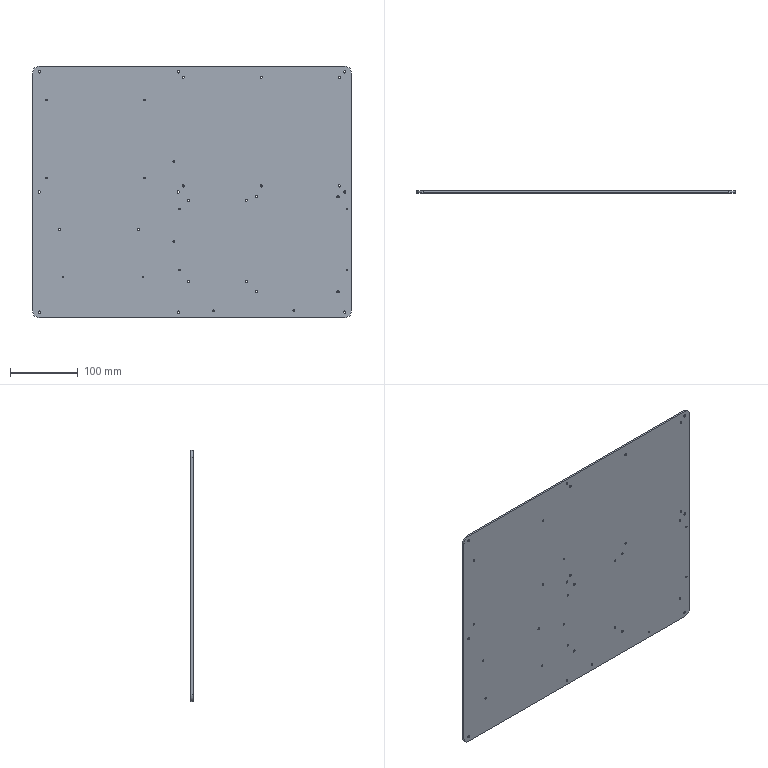CAM job | Mastercam | mm | 4 operations | part box 470 x 3 x 370
1. Contour (Ramp) | 6 - 6 平铣刀
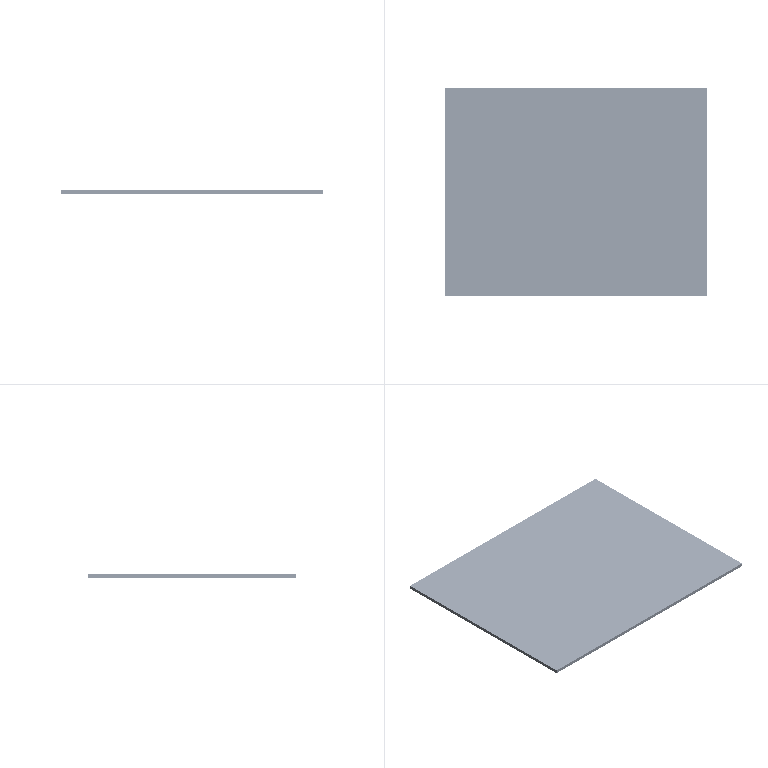2. Contour (2D) | 6 - 6 平铣刀
3. Contour (2D chamfer) | 7 - 6 倒角刀
4. Drill/Counterbore | 7 - 6 倒角刀